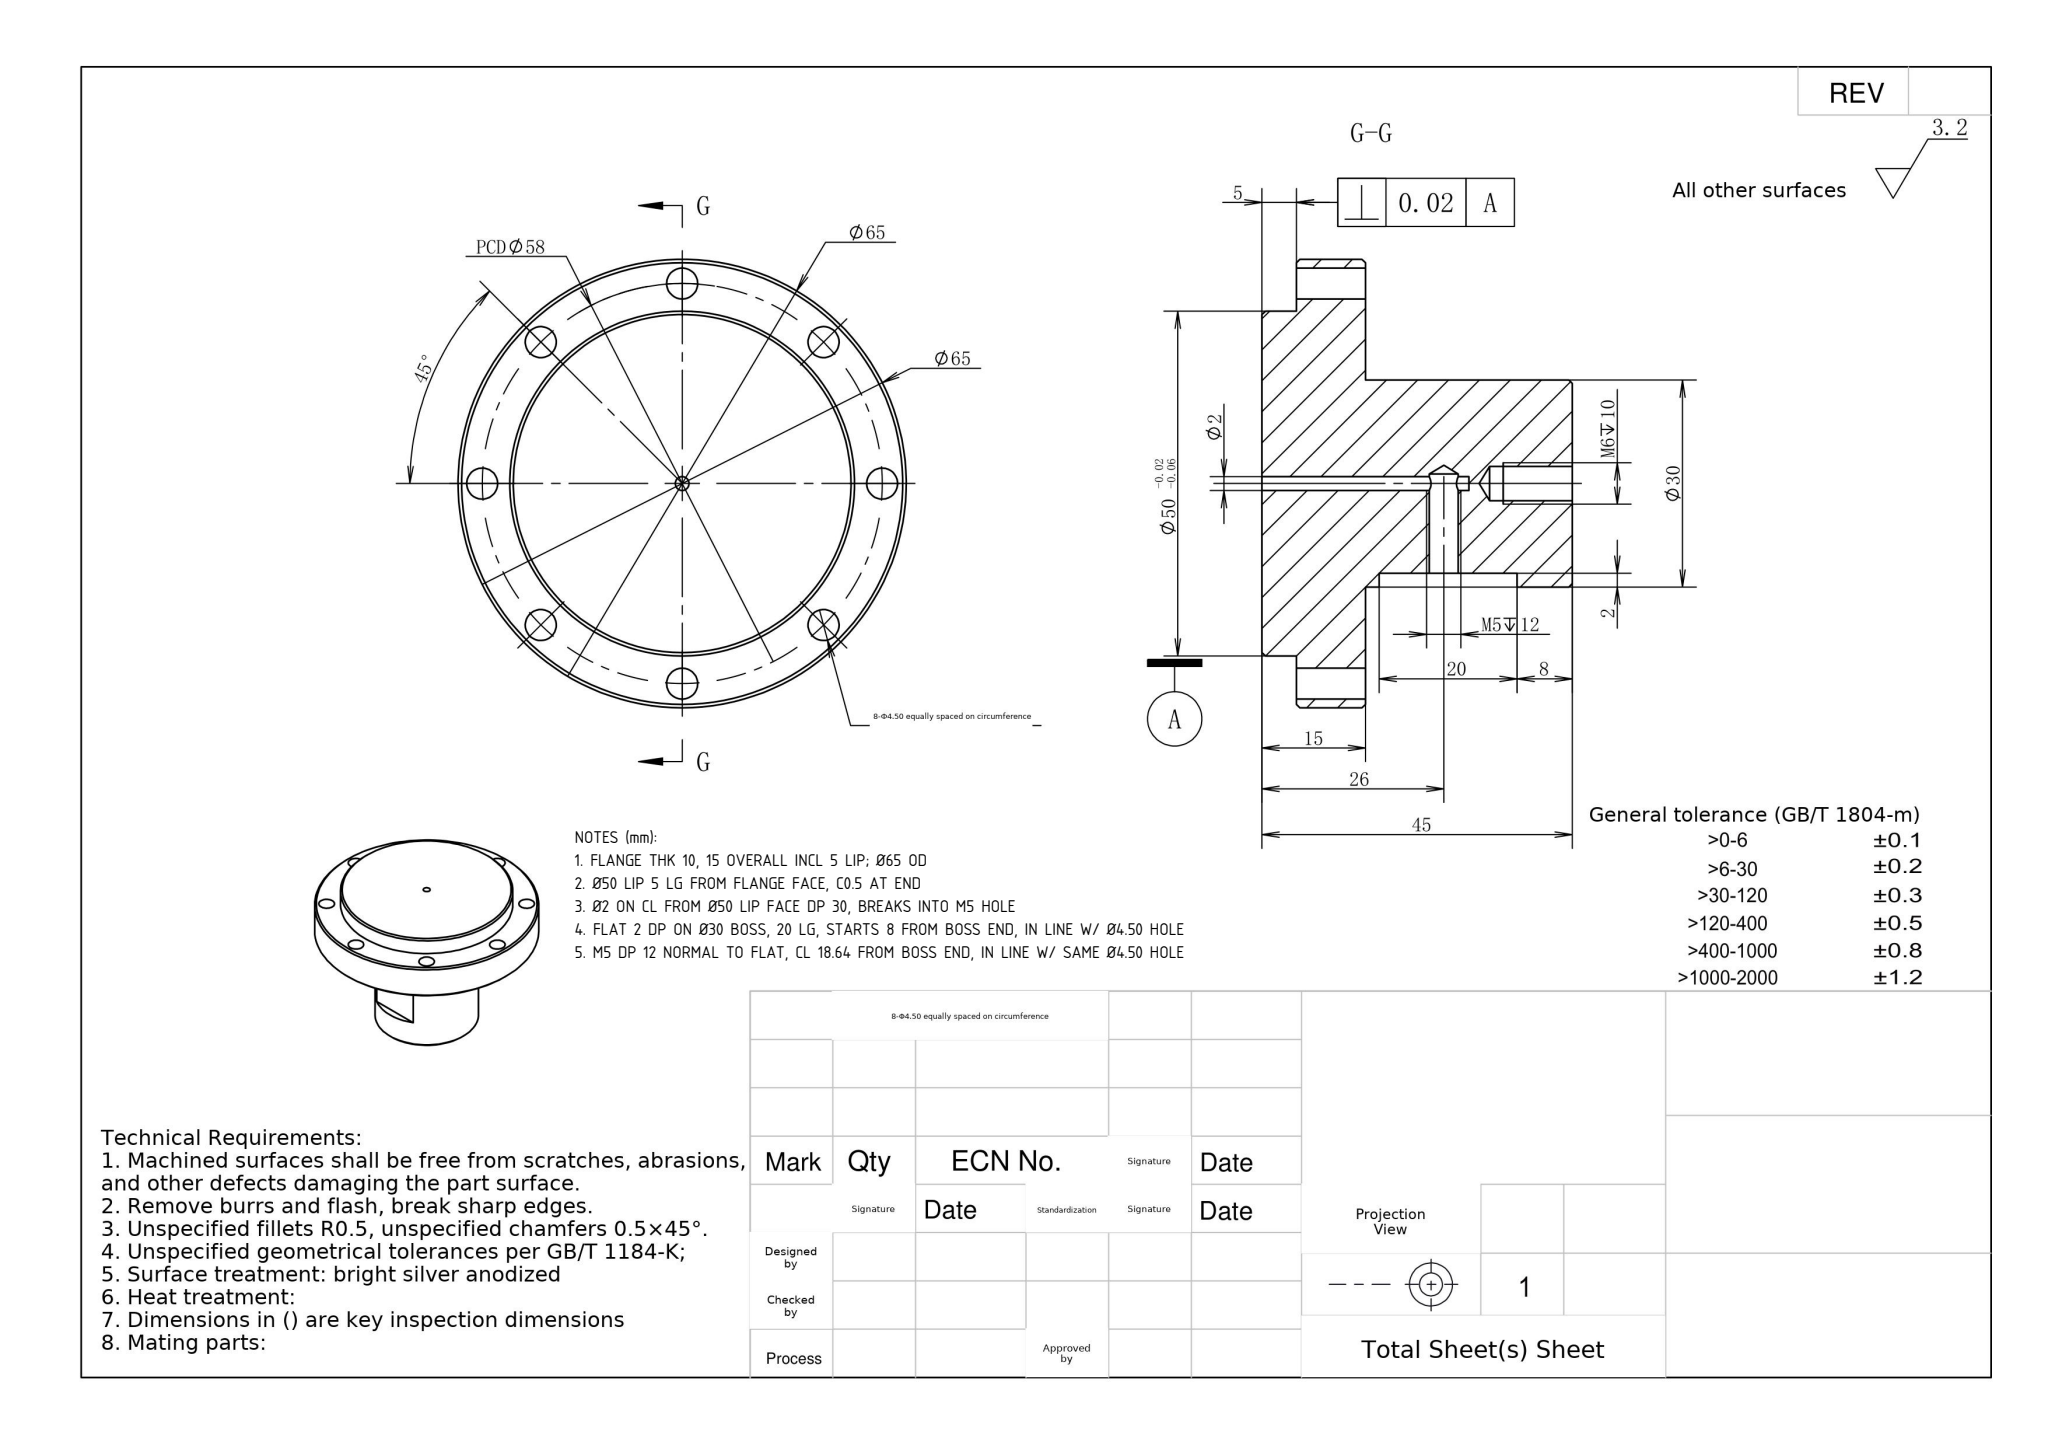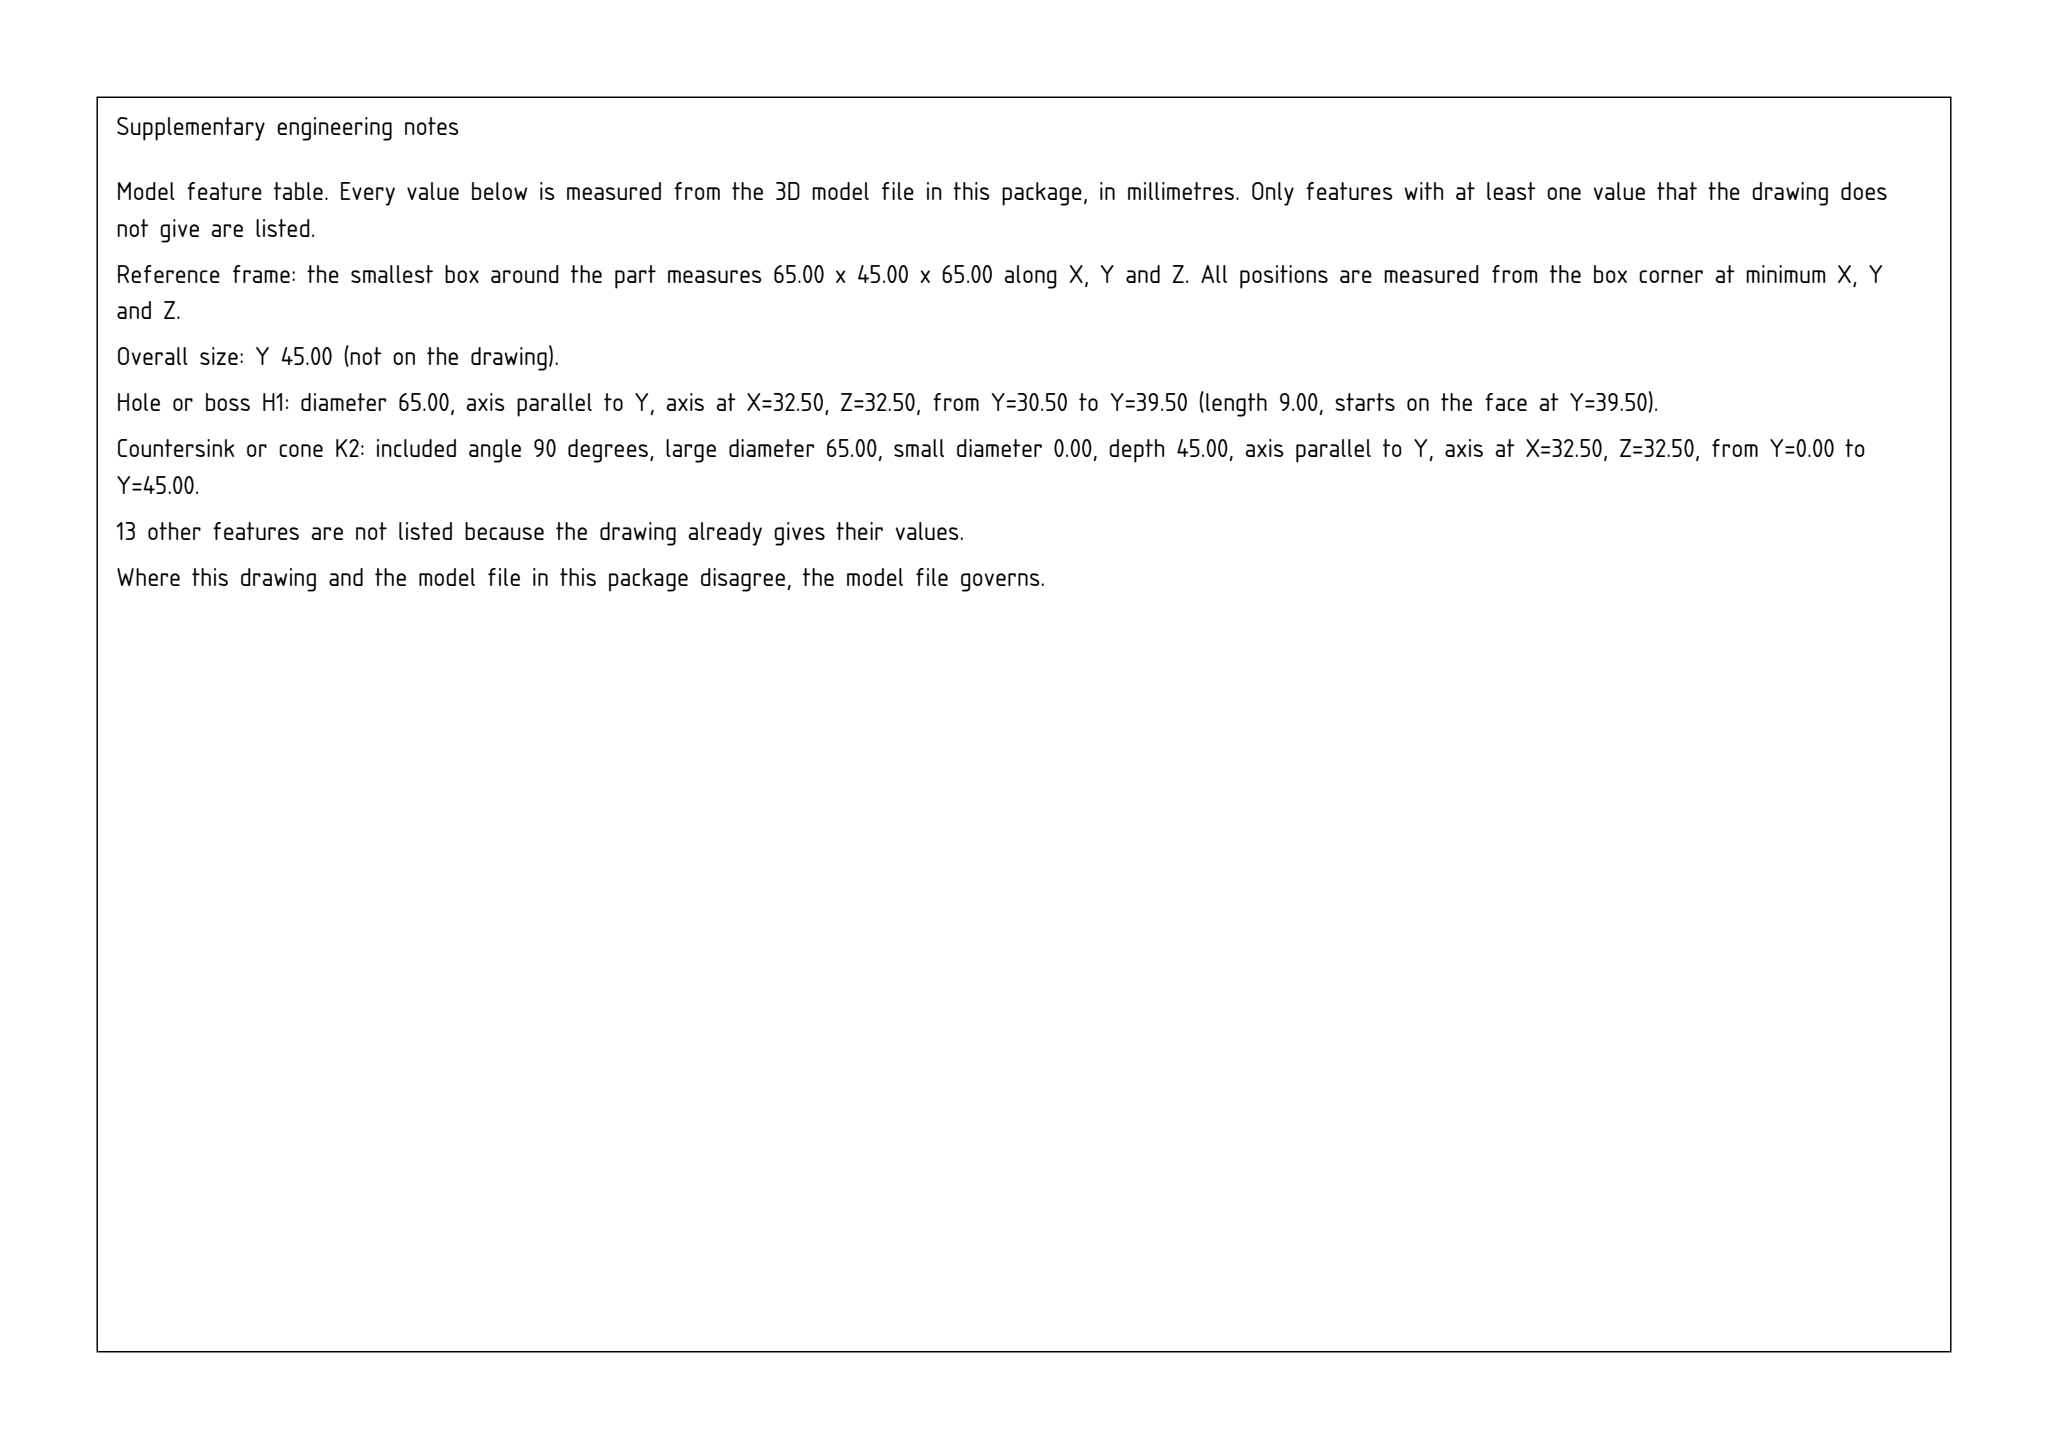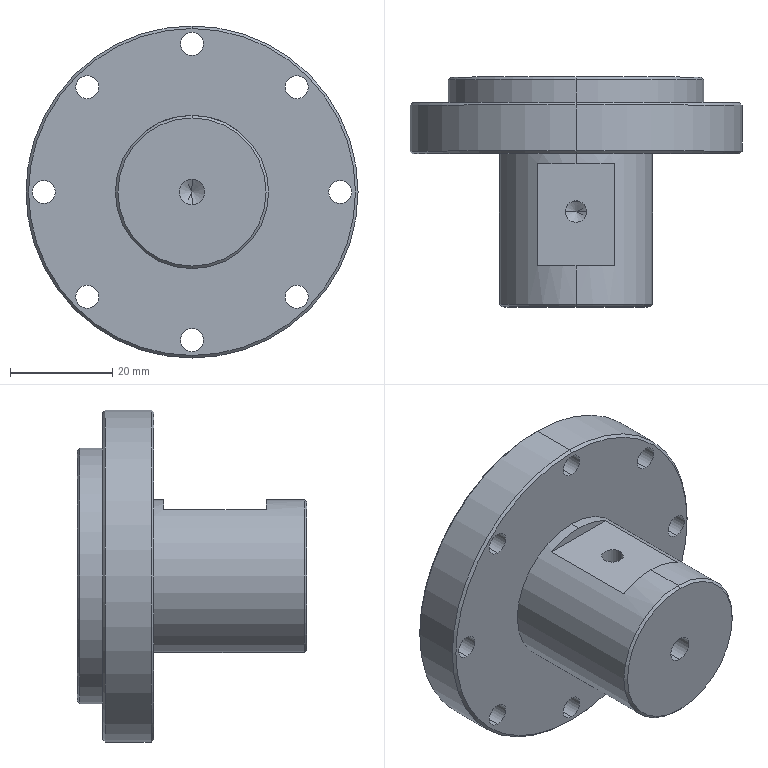Part | SolidWorks | mm | 1 solid | 50 faces | box 65 x 45 x 65 mm | volume 61915 mm3 | cylinder 30 | cone 12 | plane 8 | commonest cylinder face diameters 4.5 x16 2 x4 5 x2 4.2 x2 30 x2 50 x2 65 x2
Drawing notes:
FLANGE THK 10, 15 OVERALL INCL 5 LIP; Ø65 OD | from the solid: Ø65 cyl L=9.0 + 0.5 chamfers between y-planes 30 and 40; lip face y=45
Ø50 LIP 5 LG FROM FLANGE FACE, C0.5 AT END | from the solid: Ø50 cyl L=4.5 y=40..44.5, 90° cone ref dia 49 at y=45; flange face y=40
Ø2 ON CL FROM Ø50 LIP FACE DP 30, BREAKS INTO M5 HOLE | from the solid: Ø2 cyls L=24.51 (y=45..20.49) + L=1.79 (16.79..15.0) coaxial; gap = Ø4.2 cross hole; depth 45-15=30
FLAT 2 DP ON Ø30 BOSS, 20 LG, STARTS 8 FROM BOSS END, IN LINE W/ Ø4.50 HOLE | from the solid: Plane z=45.5 (13 from axis = 2 deep) bounded y=8..28; Ø4.50 hole at (32.5,61.5) on same +Z CL
M5 DP 12 NORMAL TO FLAT, CL 18.64 FROM BOSS END, IN LINE W/ SAME Ø4.50 HOLE | from the solid: Ø4.2 z-axis drill at x=32.5, y=18.64, LG 14.4 from flat z=45.5; boss end face y=0
build123d program:
from build123d import *

# Parameters (mm, degrees)
SKETCH1_R             = 32.5
EXTRUDE1_DEPTH        = 30
SKETCH2_R             = 36.056
SKETCH2_R_2           = 25
CUT_EXTRUDE1_DEPTH    = 5
SKETCH3_R             = 38.736
SKETCH3_R_2           = 15
CUT_EXTRUDE2_DEPTH    = 15
SKETCH4_R             = 2.25
CUT_EXTRUDE3_DEPTH    = 53.321
CIRPATTERN1_COUNT     = 8
SKETCH5_R             = 1
EXTRUDE2_DEPTH        = 40
EXTRUDE3_START        = 15
SKETCH6_R             = 15
EXTRUDE3_DEPTH        = 15
SKETCH7_W             = 2
SKETCH7_H             = 20
EXTRUDE4_DEPTH        = 7.5
M5_TAPPED_HOLE1_D     = 4.2
M5_TAPPED_HOLE1_DEPTH = 14.4
M5_TAPPED_HOLE1_TIP   = 1.262
M6_TAPPED_HOLE1_D     = 5
M6_TAPPED_HOLE1_DEPTH = 12
M6_TAPPED_HOLE1_TIP   = 1.502
CHAMFER1_SIZE         = 0.5


with BuildPart() as part:
    # Sketch1 → Extrude1 (new body)
    with BuildSketch(Plane(origin=(0, 0, 0), x_dir=(1, 0, 0), z_dir=(0, 1, 0))):
        with Locations(Location((0, 0, 0), (0, 0, 270))):
            Circle(SKETCH1_R)
    extrude(amount=EXTRUDE1_DEPTH)

    # Sketch2 → Cut-Extrude1 (cut)
    with BuildSketch(Plane(origin=(0, 30, 0), x_dir=(1, 0, 0), z_dir=(0, 1, 0))):
        Circle(SKETCH2_R)
        with Locations(Location((0, 0, 0), (0, 0, 270))):
            Circle(SKETCH2_R_2, mode=Mode.SUBTRACT)
    extrude(amount=-CUT_EXTRUDE1_DEPTH, mode=Mode.SUBTRACT)

    # Sketch3 → Cut-Extrude2 (cut)
    with BuildSketch(Plane.XZ):
        Circle(SKETCH3_R)
        with Locations(Location((0, 0, 0), (0, 0, 270))):
            Circle(SKETCH3_R_2, mode=Mode.SUBTRACT)
    extrude(amount=-CUT_EXTRUDE2_DEPTH, mode=Mode.SUBTRACT)

    # Sketch4 → Cut-Extrude3 (cut, through all)
    with BuildSketch(Plane(origin=(0, 25, 0), x_dir=(1, 0, 0), z_dir=(0, 1, 0))):
        with Locations(Location((0, 29, 0), (0, 0, 270))):
            Circle(SKETCH4_R)
    cut_extrude3 = extrude(amount=-CUT_EXTRUDE3_DEPTH, mode=Mode.SUBTRACT)

    # CirPattern1: Cut-Extrude3 ×8 about axis
    cirpattern1_axis = Axis((0, 0, 0), (0, 1, 0))
    for i in range(1, CIRPATTERN1_COUNT):
        add(cut_extrude3.rotate(cirpattern1_axis, i * 360 / CIRPATTERN1_COUNT), mode=Mode.SUBTRACT)

    # Sketch5 → Extrude2 (cut)
    with BuildSketch(Plane(origin=(0, 30, 0), x_dir=(1, 0, 0), z_dir=(0, 1, 0))):
        with Locations(Location((0, 0, 0), (0, 0, 270))):
            Circle(SKETCH5_R)
    extrude(amount=-EXTRUDE2_DEPTH, mode=Mode.SUBTRACT)

    # Sketch6 → Extrude3 (add)
    with BuildSketch(Plane.XZ.offset(EXTRUDE3_START)):
        with Locations(Location((0, 0, 0), (0, 0, 270))):
            Circle(SKETCH6_R)
    extrude(amount=-EXTRUDE3_DEPTH)

    # Sketch7 → Extrude4 (cut, symmetric)
    with BuildSketch(Plane(origin=(0, 0, 0), x_dir=(0, 0, -1), z_dir=(1, 0, 0))):
        with Locations((-14, 3)):
            Rectangle(SKETCH7_W, SKETCH7_H)
    extrude(amount=EXTRUDE4_DEPTH, both=True, mode=Mode.SUBTRACT)

    # M5 Tapped Hole1
    with Locations(Plane.XY.offset(13)):
        with Locations((0, 3.64)):
            Hole(M5_TAPPED_HOLE1_D / 2, depth=M5_TAPPED_HOLE1_DEPTH)
            with Locations((0, 0, -(M5_TAPPED_HOLE1_DEPTH + M5_TAPPED_HOLE1_TIP / 2))):  # 118° drill point
                Cone(0, M5_TAPPED_HOLE1_D / 2, M5_TAPPED_HOLE1_TIP, mode=Mode.SUBTRACT)

    # M6 Tapped Hole1
    with Locations(Plane(origin=(0, -15, 0), x_dir=(-1, 0, 0), z_dir=(0, -1, 0))):
        with Locations((0, 0)):
            Hole(M6_TAPPED_HOLE1_D / 2, depth=M6_TAPPED_HOLE1_DEPTH)
            with Locations((0, 0, -(M6_TAPPED_HOLE1_DEPTH + M6_TAPPED_HOLE1_TIP / 2))):  # 118° drill point
                Cone(0, M6_TAPPED_HOLE1_D / 2, M6_TAPPED_HOLE1_TIP, mode=Mode.SUBTRACT)

    # Chamfer1
    chamfer1_edges = [part.edges().sort_by_distance(p)[0] for p in [
        (0, 15, -32.5),
        (0, -15, 15),
        (0, 25, -32.5),
        (0, 30, -25),
    ]]
    chamfer(chamfer1_edges, length=CHAMFER1_SIZE)


solid = part.part